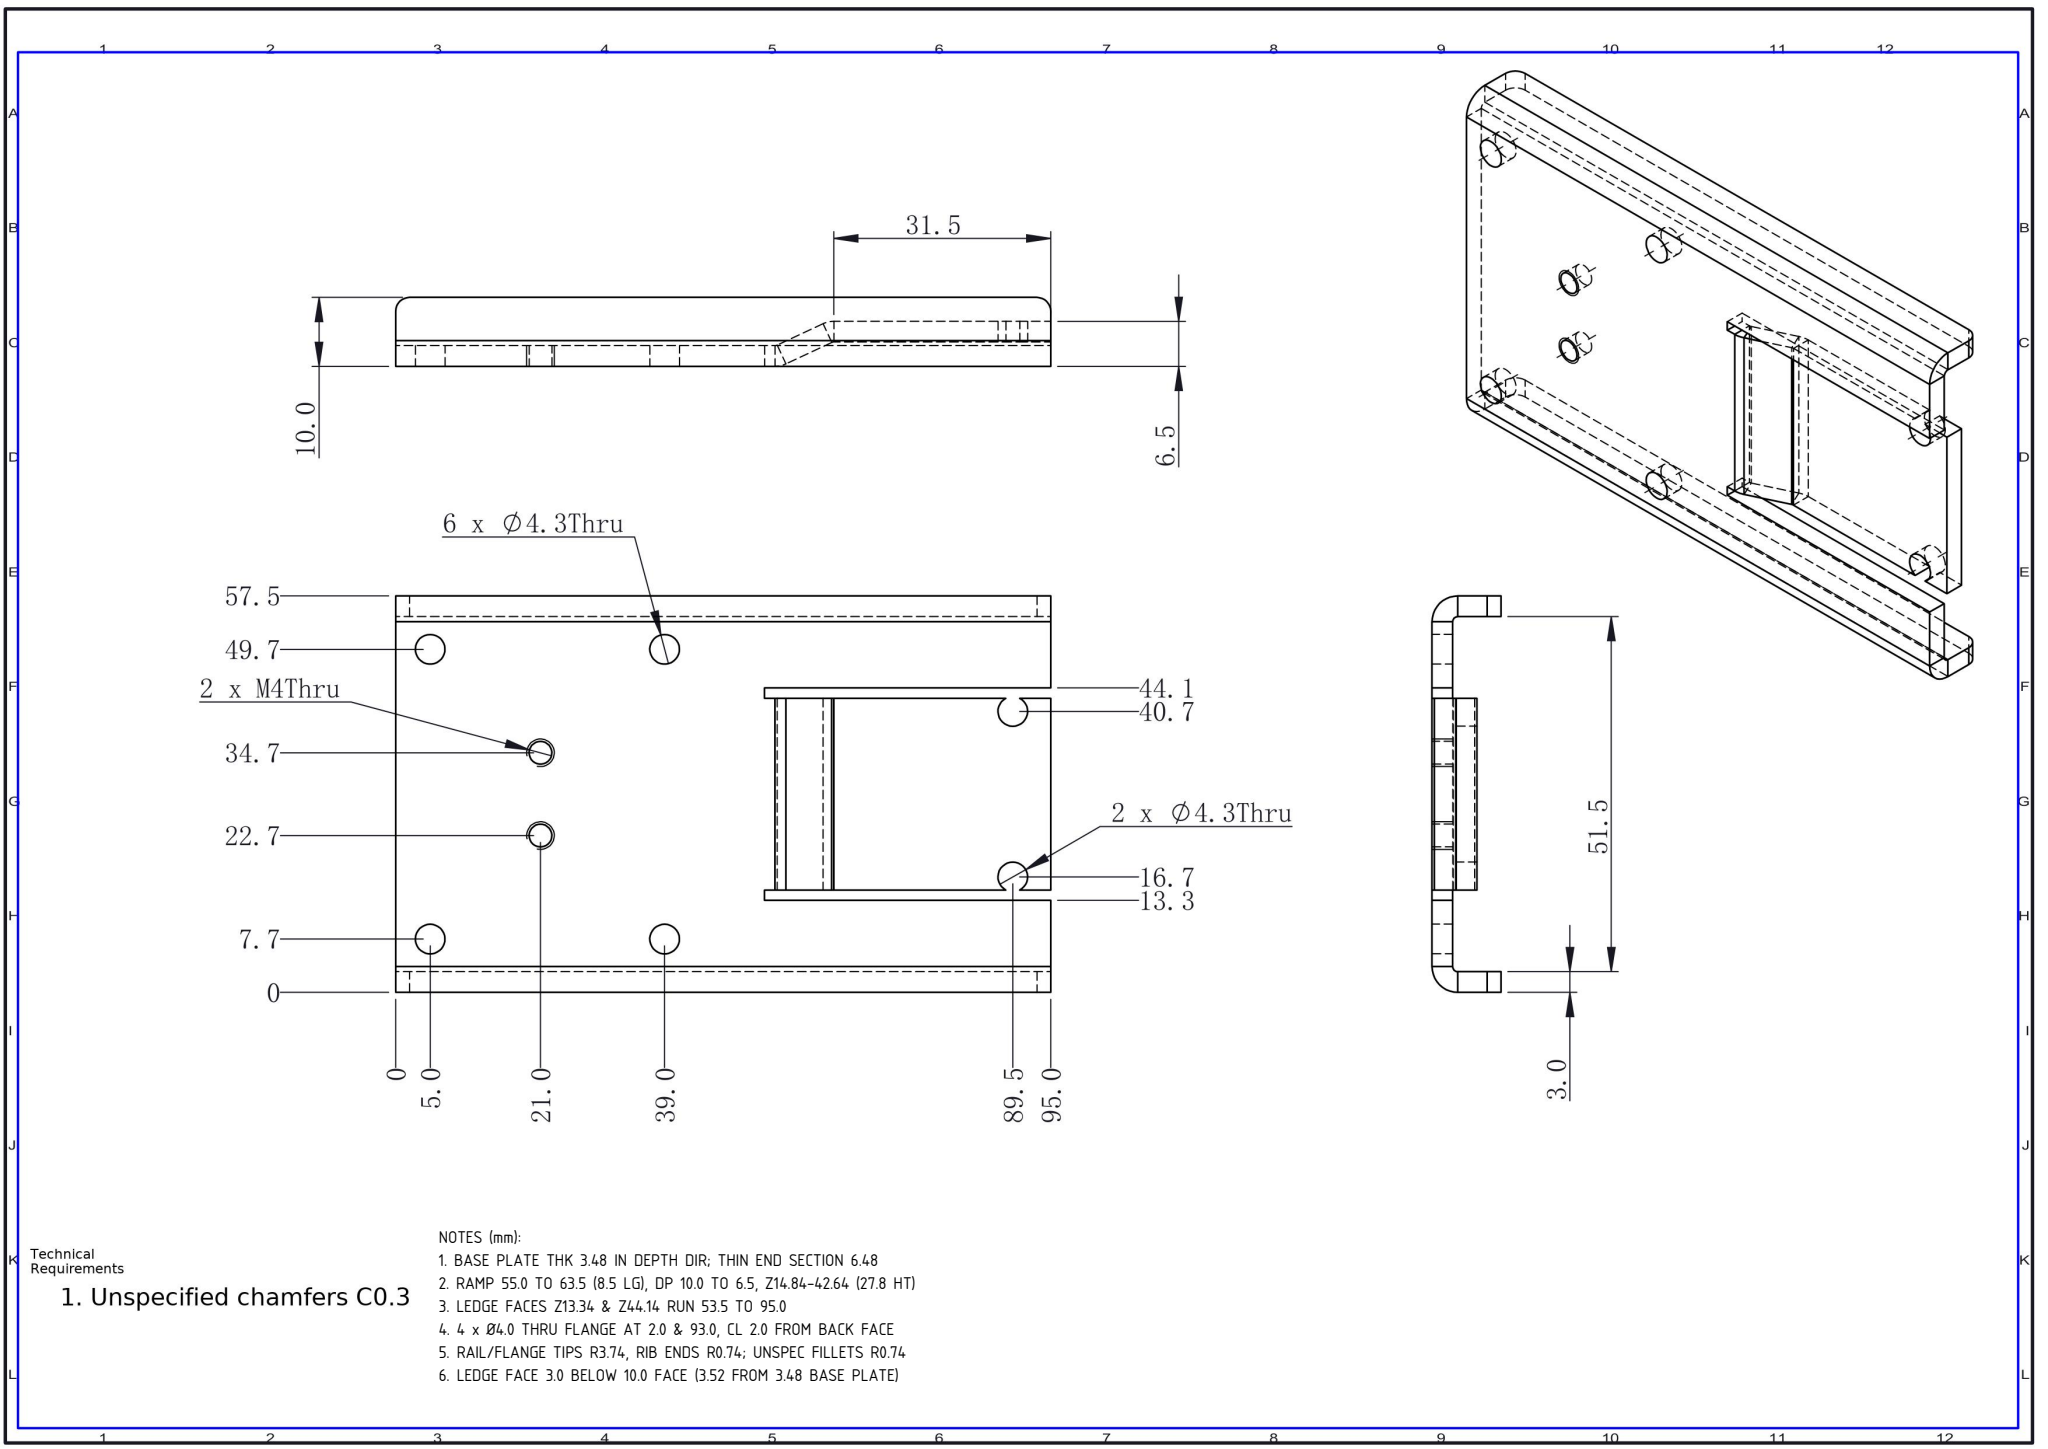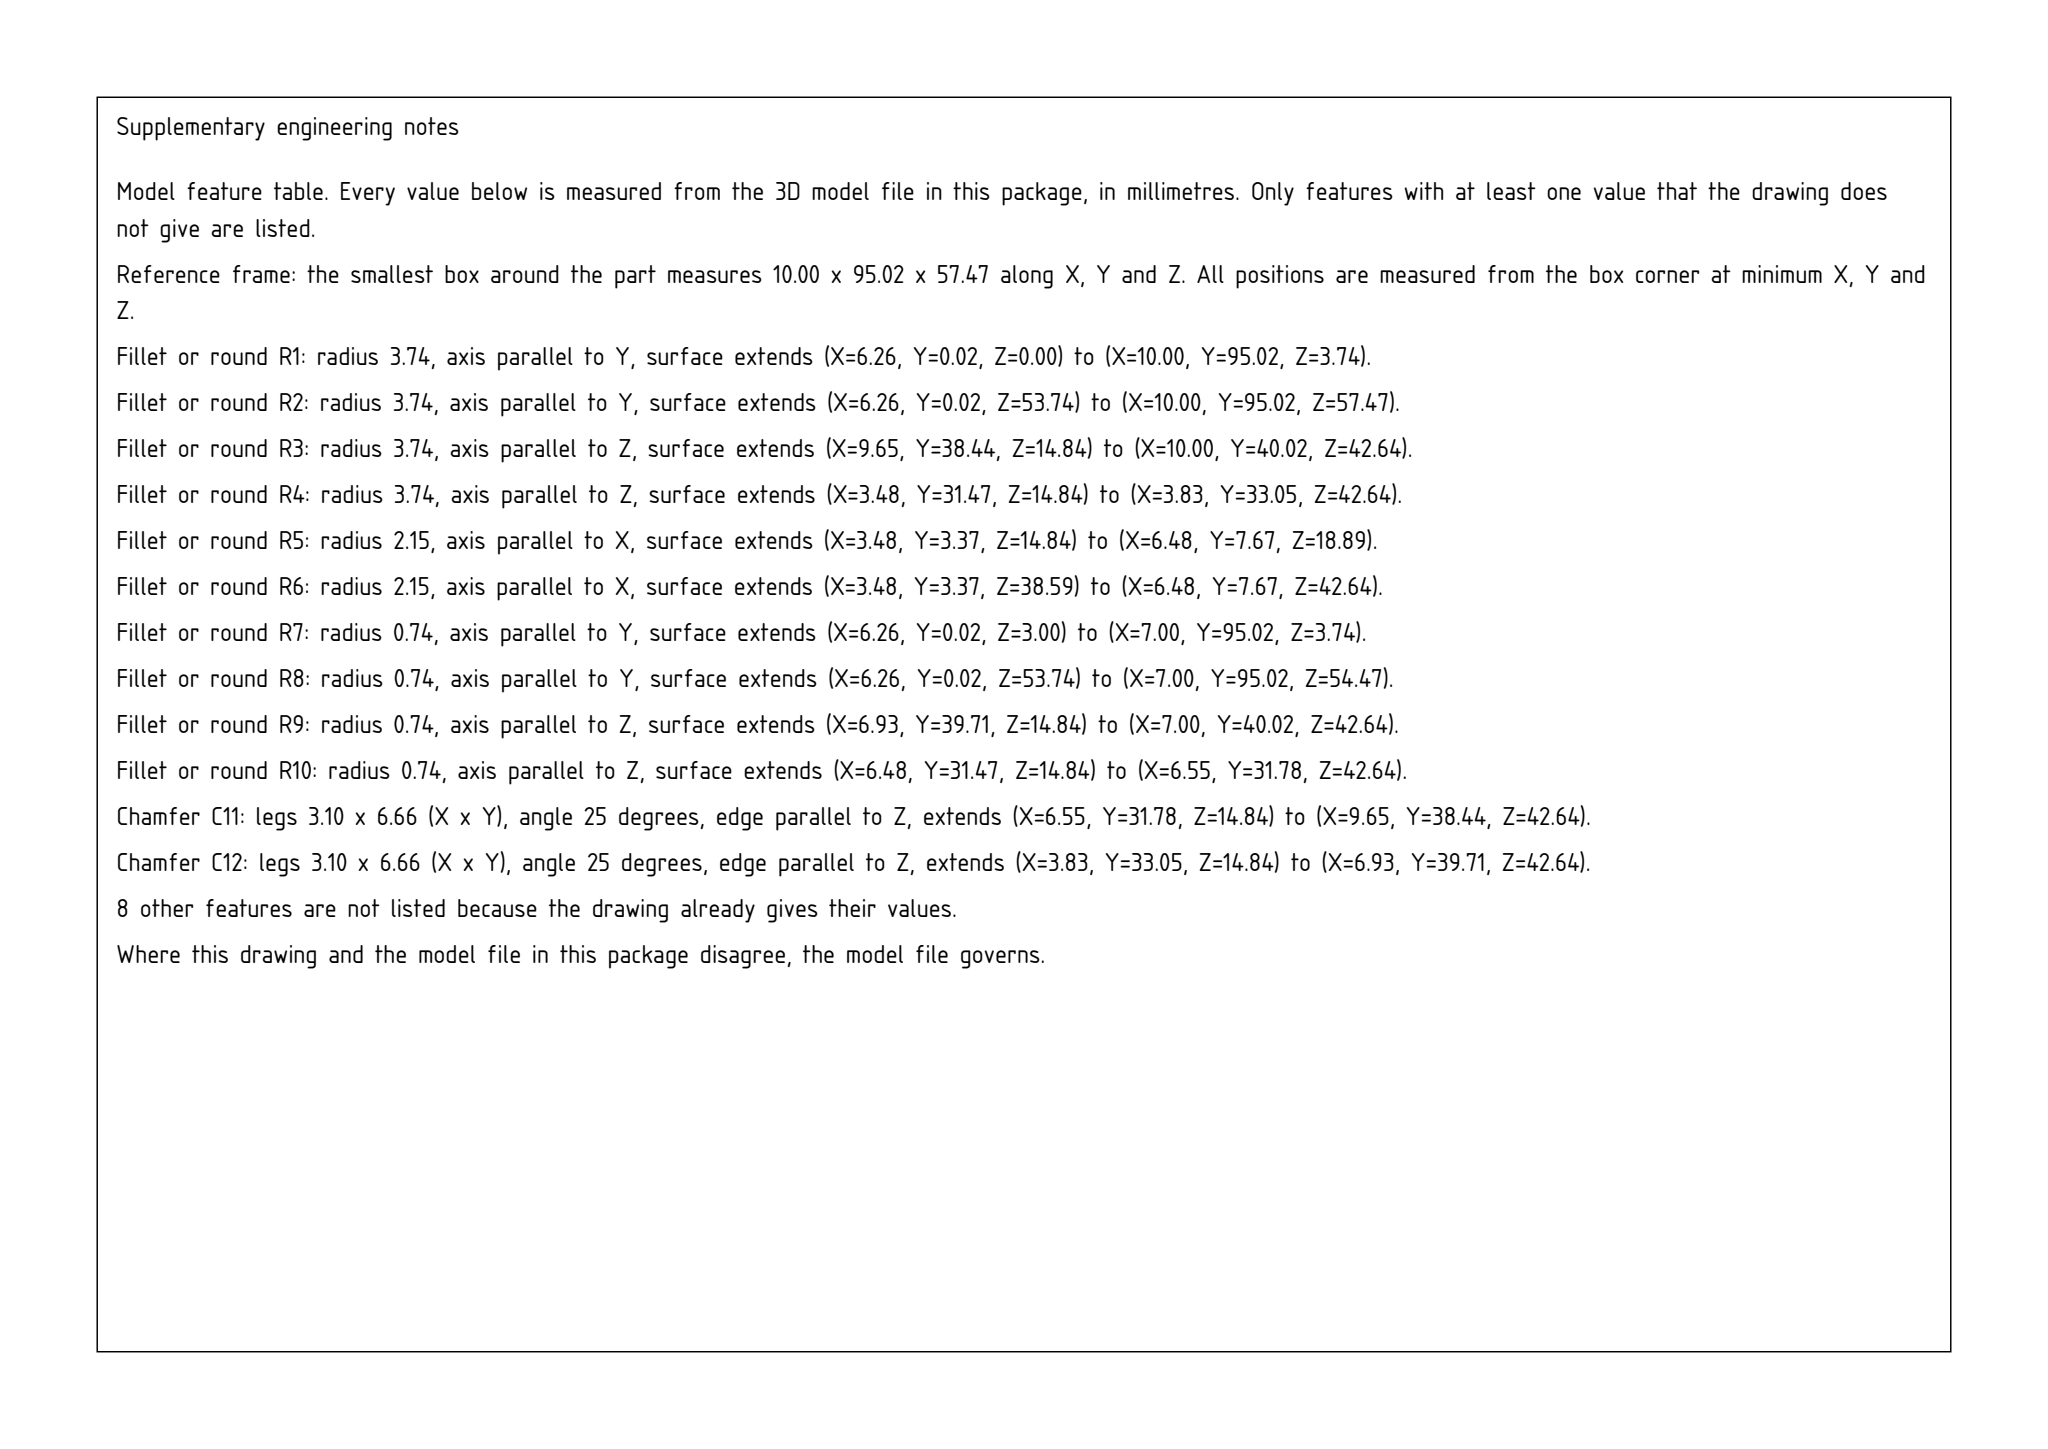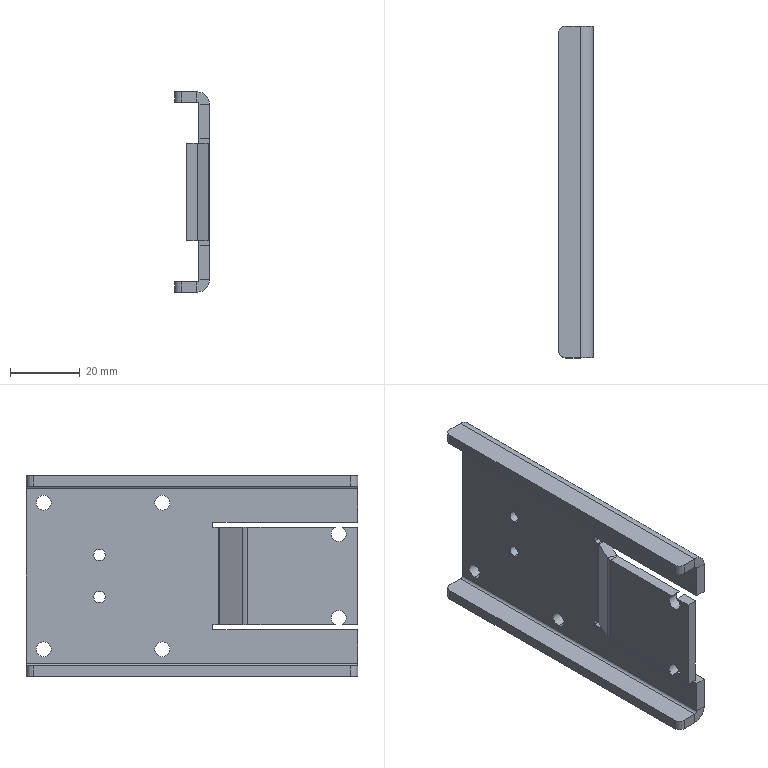Part | SolidWorks | mm | 1 solid | 67 faces | box 10 x 95.02 x 57.47 mm | volume 19192 mm3 | plane 40 | cylinder 27 | commonest cylinder face diameters 4.3 x11 3.3 x4 7.473 x4 1.473 x4 4 x4
Drawing notes:
BASE PLATE THK 3.48 IN DEPTH DIR; THIN END SECTION 6.48 | from the solid: x planes 0.0, 3.48, 6.48, 10.0; flange faces z 0-3.0
RAMP 55.0 TO 63.5 (8.5 LG), DP 10.0 TO 6.5, Z14.84-42.64 (27.8 HT) | from the solid: z-axis cyls (6.26,40.02) & (7.21,31.47) len 27.8, z planes 14.84/42.64; y_draw 55.0 & 63.55; x 10.0 to 6.48
LEDGE FACES Z13.34 & Z44.14 RUN 53.5 TO 95.0 | from the solid: y plane 41.52 (=53.5 from datum) to y 95.02; z planes 13.34 & 44.14
4 x Ø4.0 THRU FLANGE AT 2.0 & 93.0, CL 2.0 FROM BACK FACE | from the solid: cyl dia 4.0 axis z, x=2.0, y=2.02 & 93.02, len 3.0, 2 ea; y_draw=95.02-y
RAIL/FLANGE TIPS R3.74, RIB ENDS R0.74; UNSPEC FILLETS R0.74 | from the solid: cyl dia 7.473 (R3.74) y-axis at z=3.74/53.74; dia 1.473 (R0.74) rail & rib ends
LEDGE FACE 3.0 BELOW 10.0 FACE (3.52 FROM 3.48 BASE PLATE) | from the solid: X planes at 0/3.48/6.48/7.0/10.0; ledge front face offset X=7.0 -> 10.0-7.0=3.0, 7.0-3.48=3.52